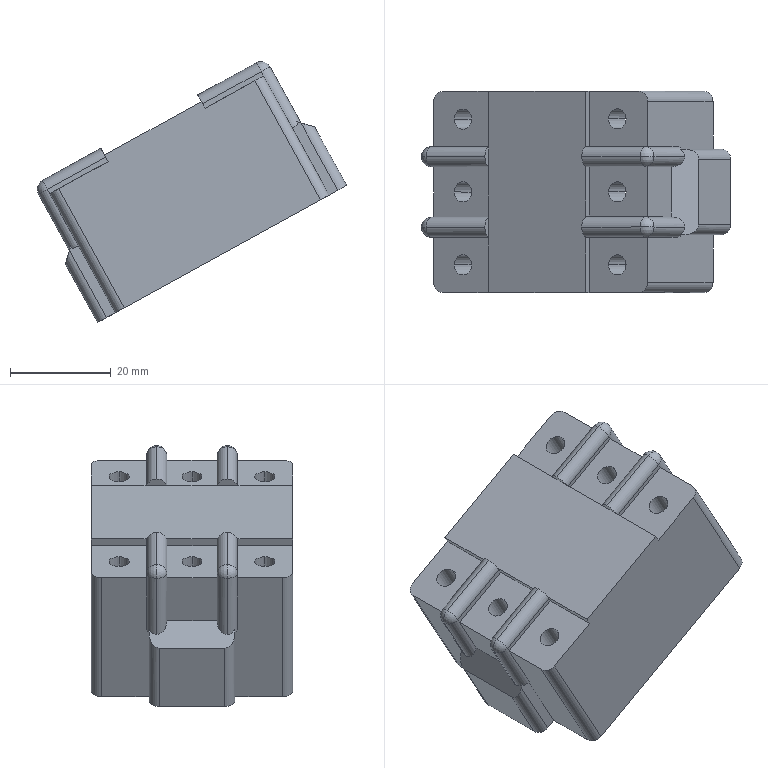Component | SolidWorks | Electrical box-1 | 1 solid | 95 faces | box 61.49 x 40 x 51.85 mm | volume 27079 mm3 | plane 51 | cylinder 36 | sphere 8 | commonest cylinder face diameters 4 x36